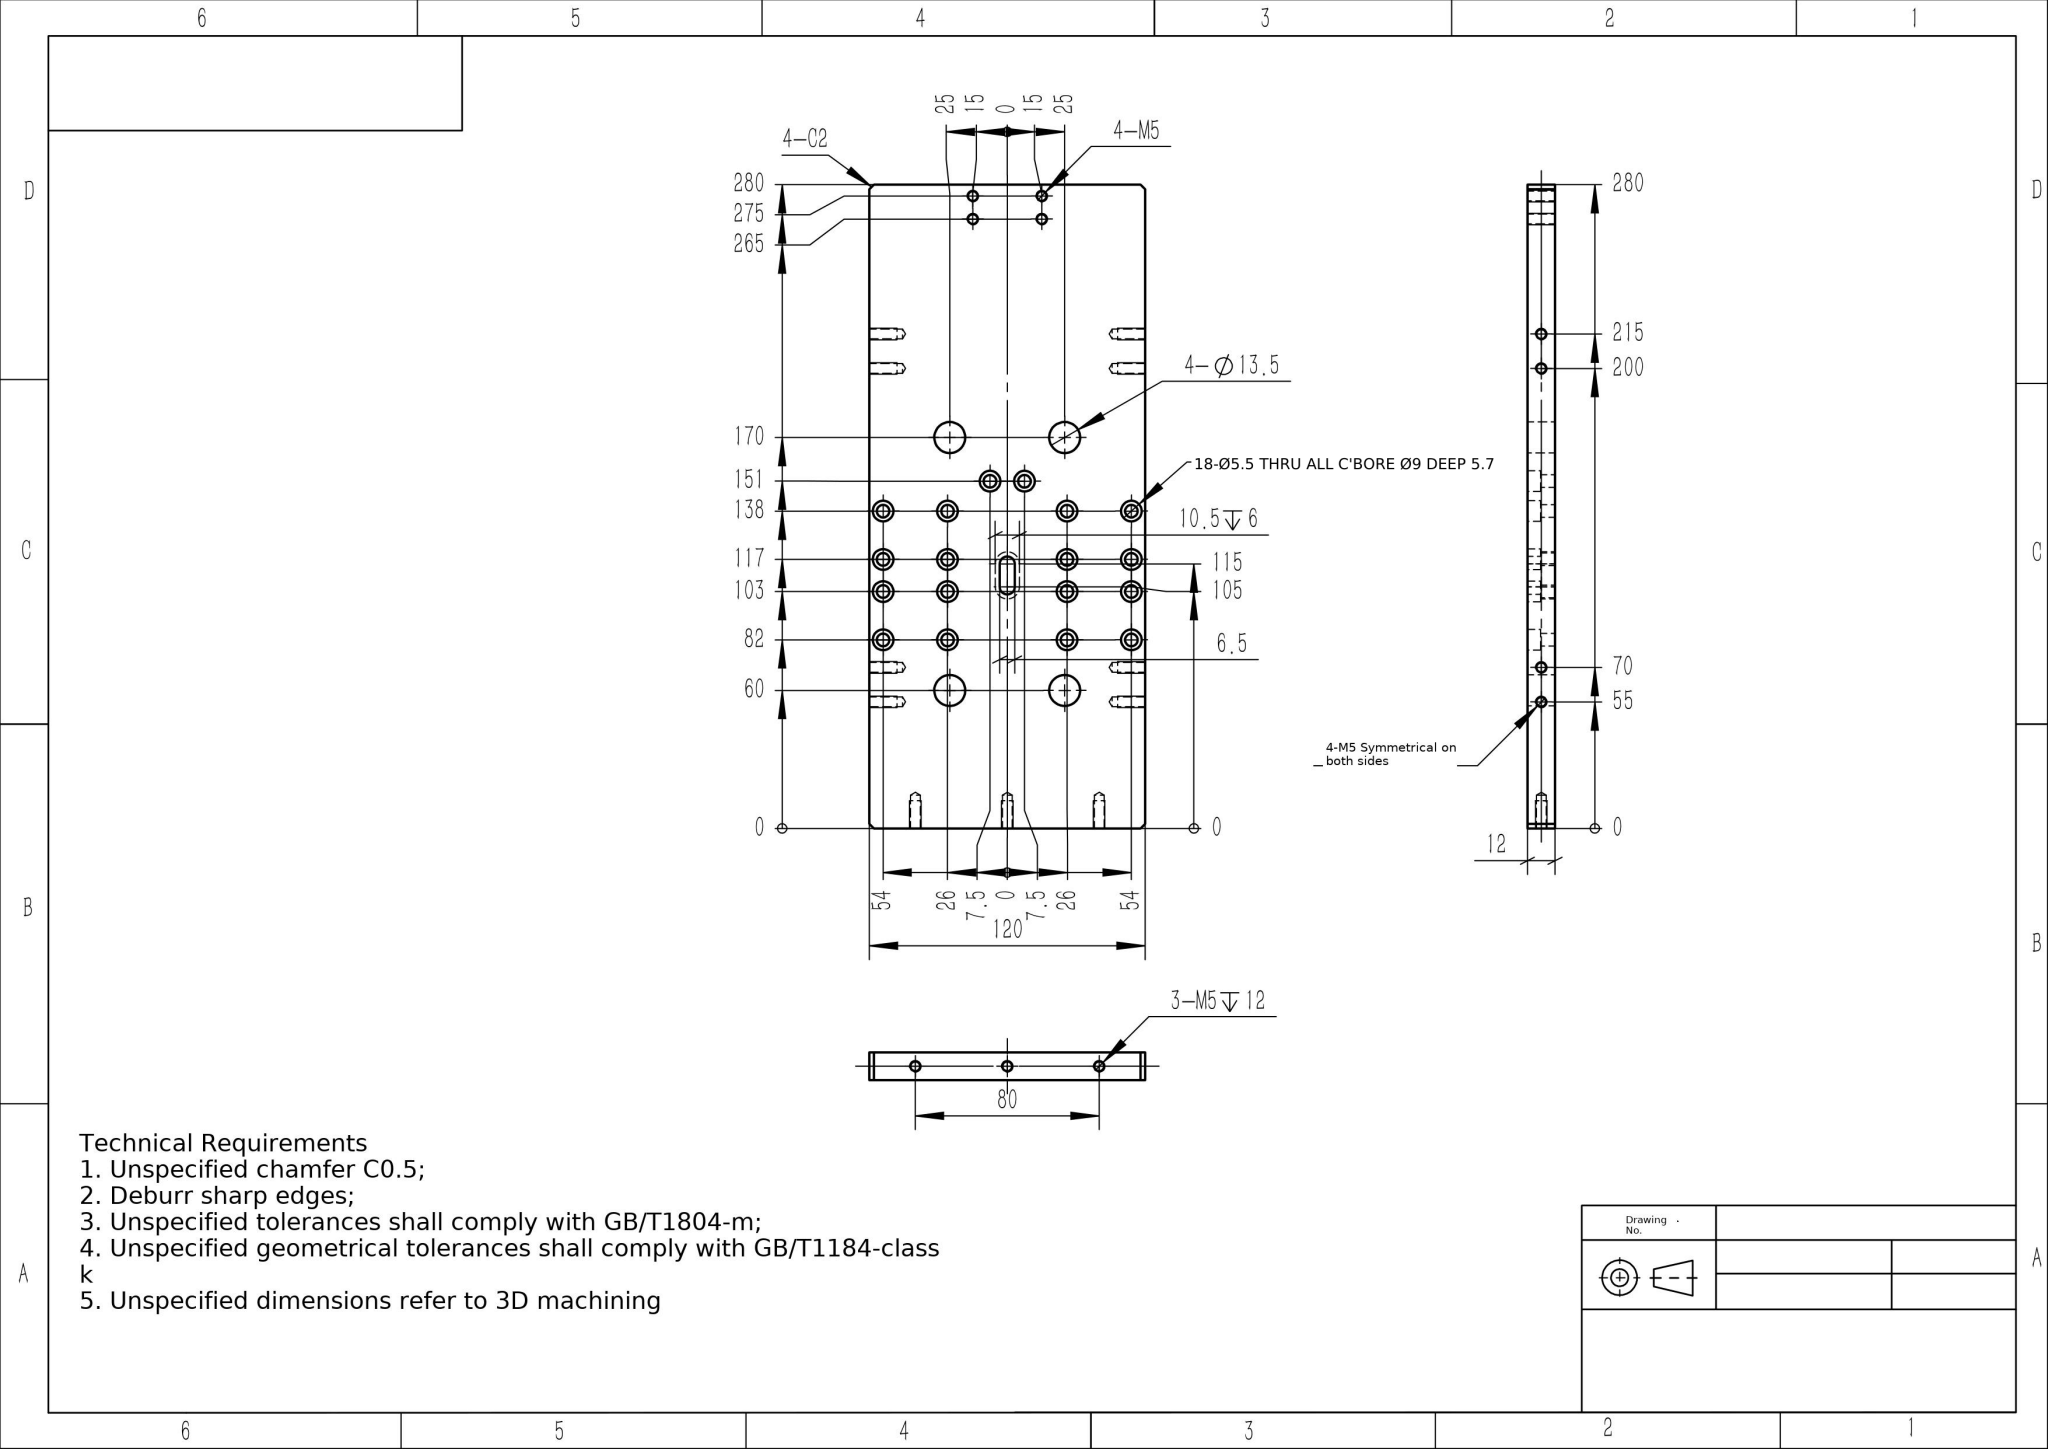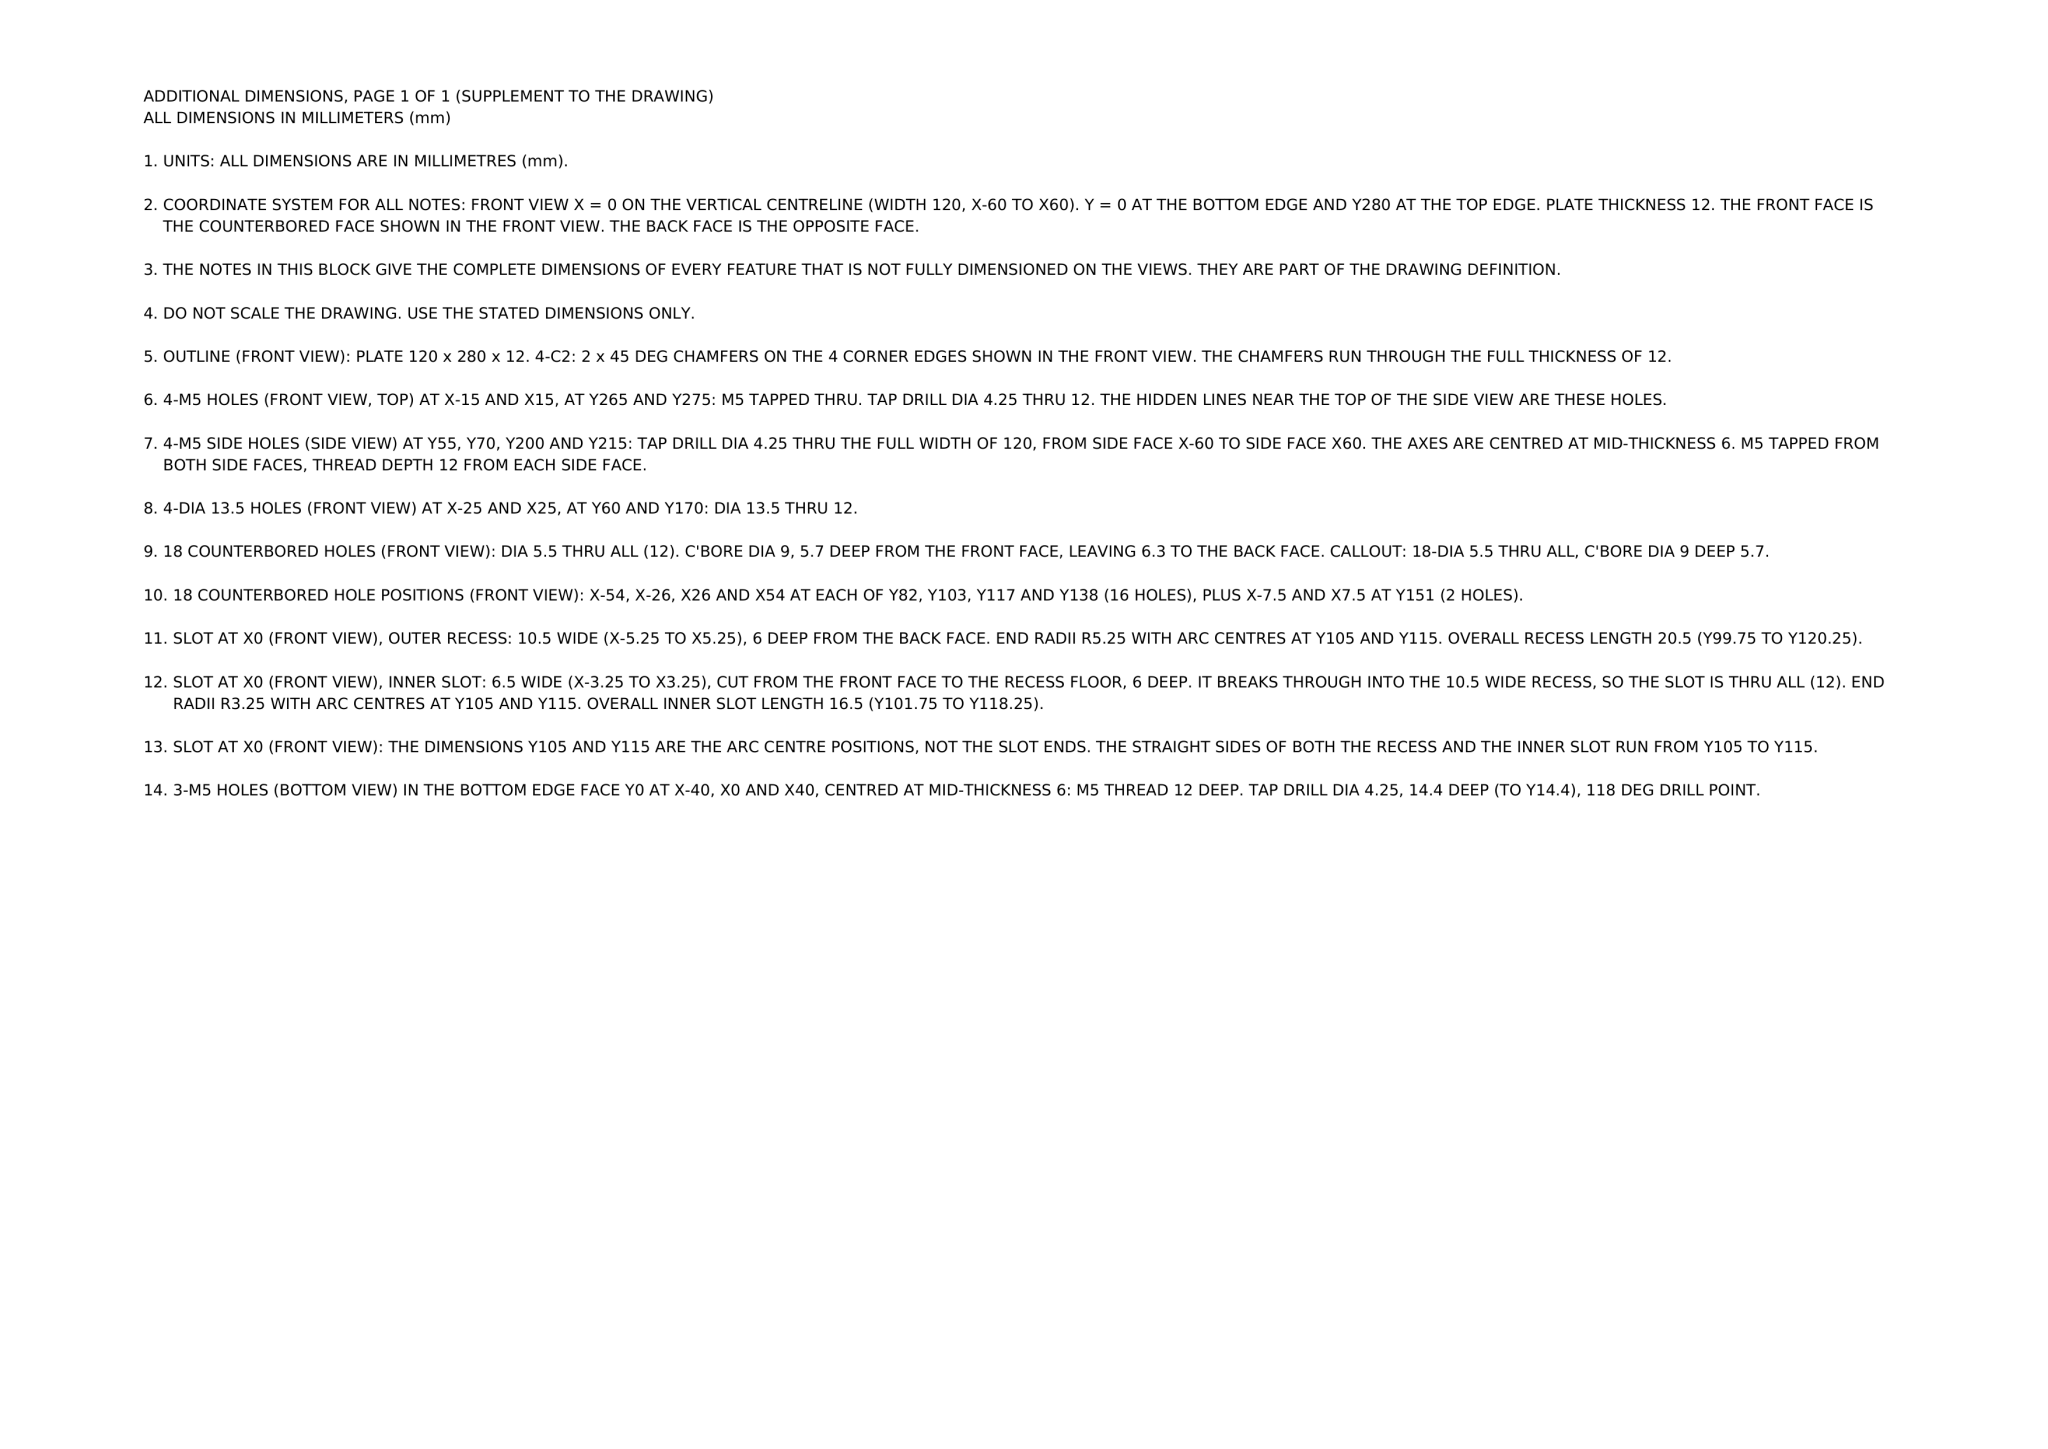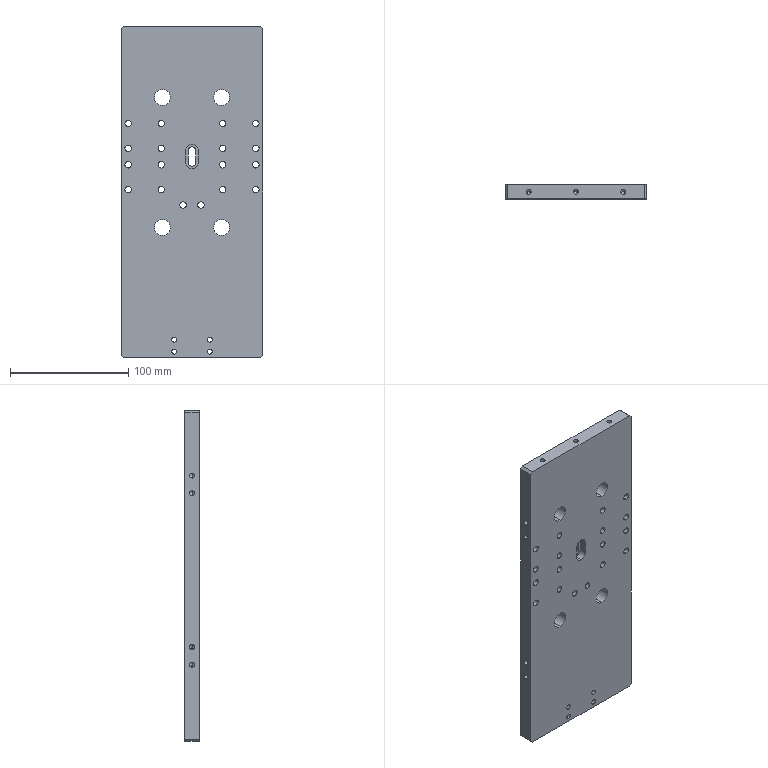Part | NX | mm | 1 solid | 171 faces | box 120 x 12 x 280 mm | volume 382279 mm3 | cylinder 116 | plane 33 | cone 22 | commonest cylinder face diameters 9 x36 5.5 x36 4.25 x30 13.5 x8 10.5 x3 6.5 x3